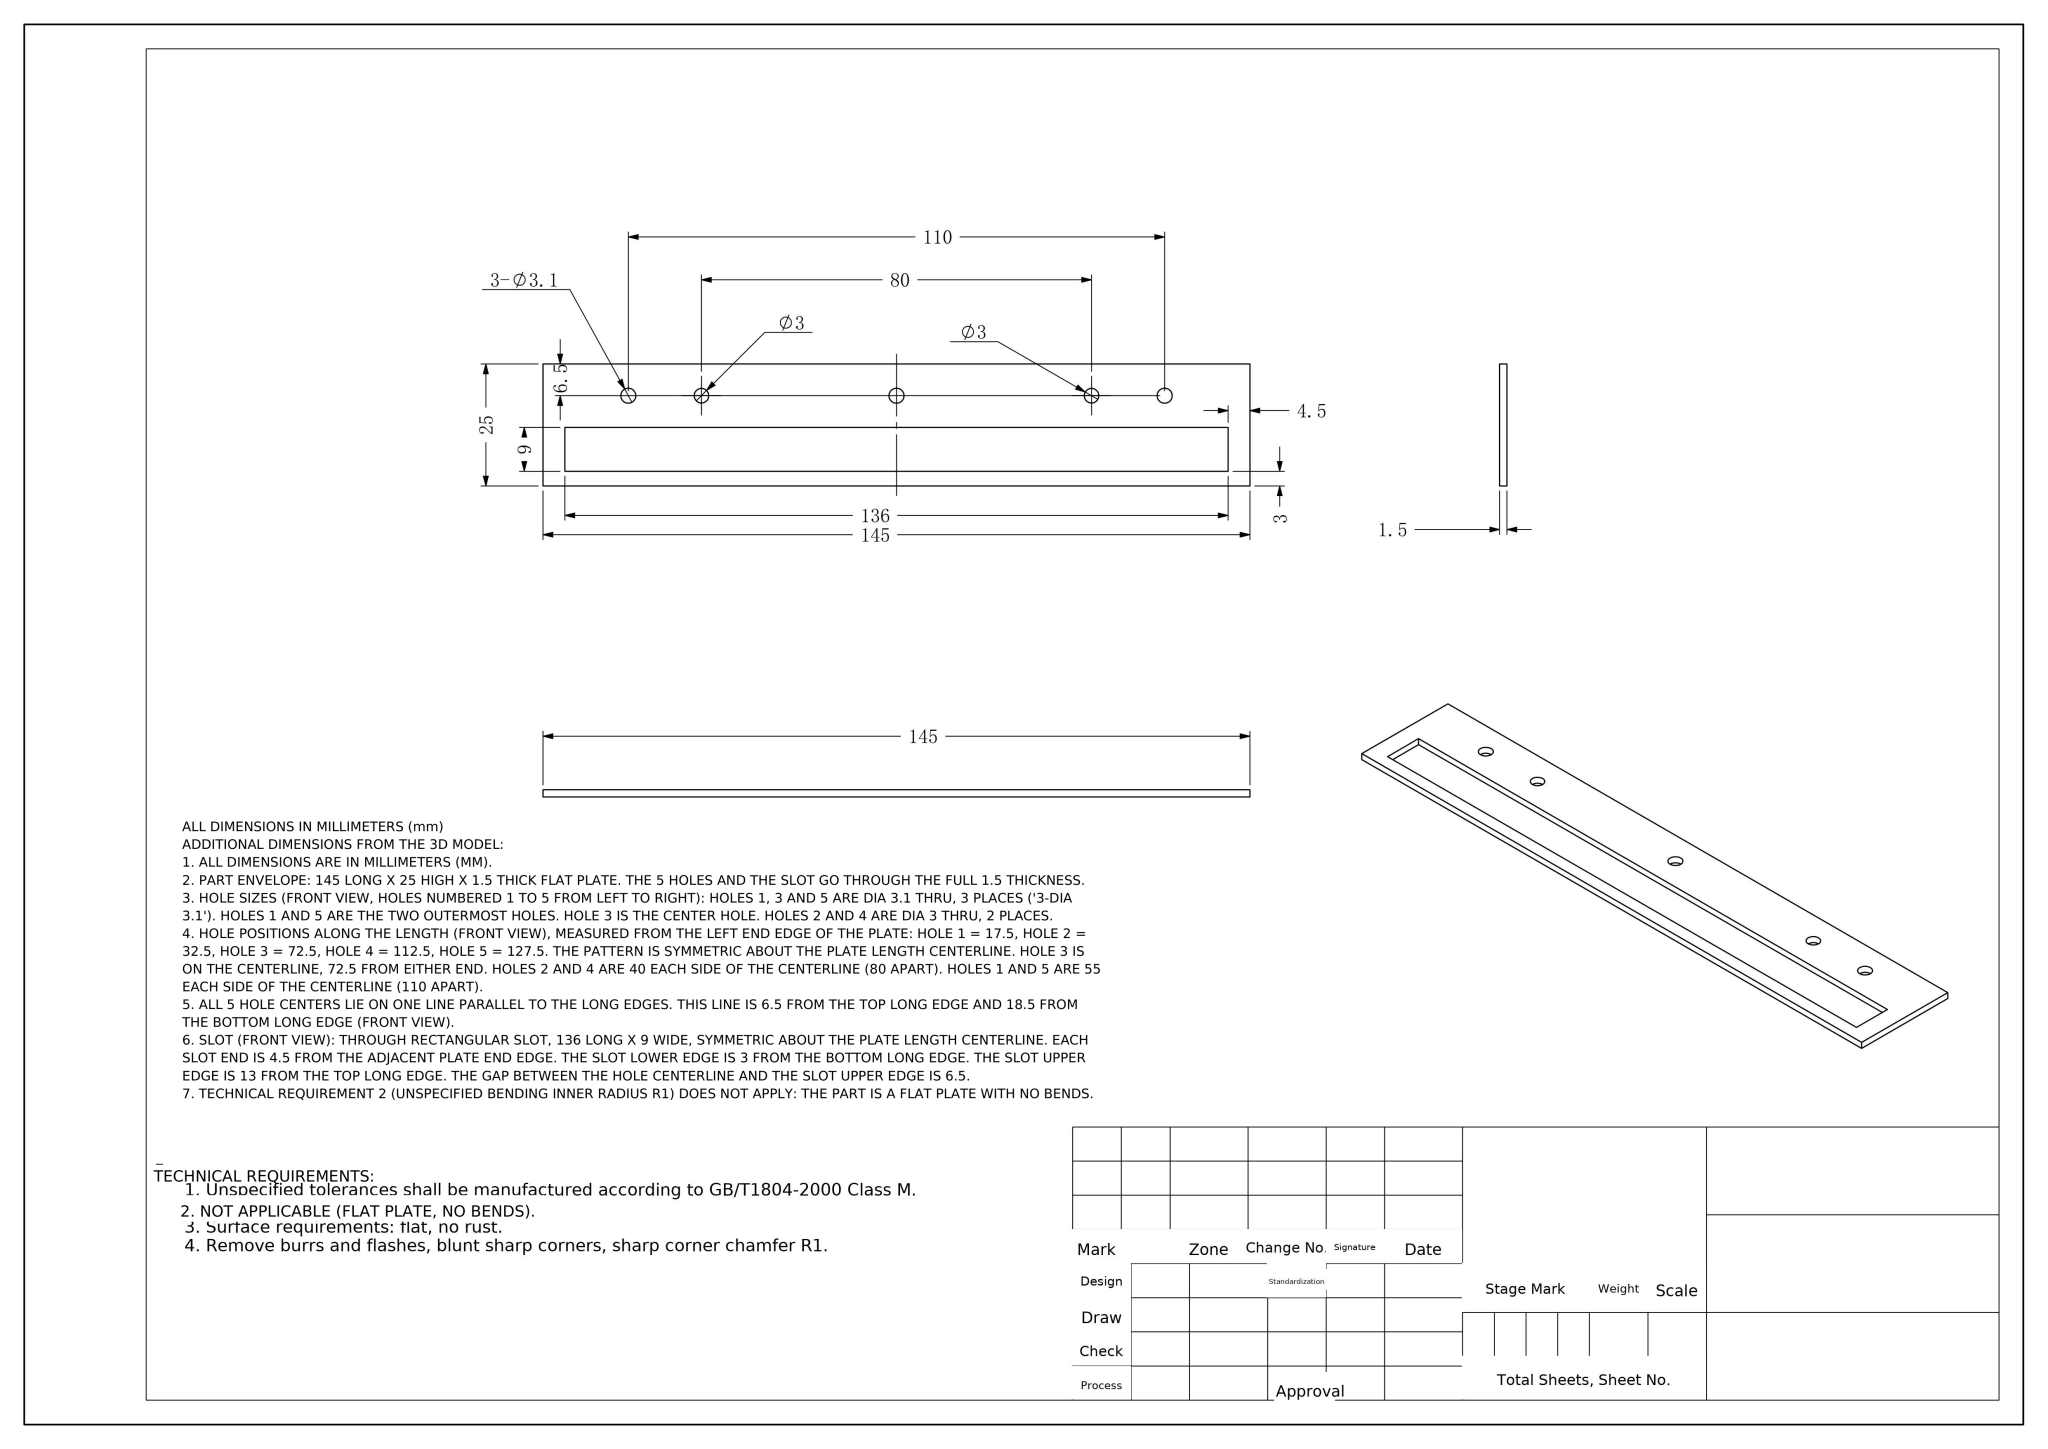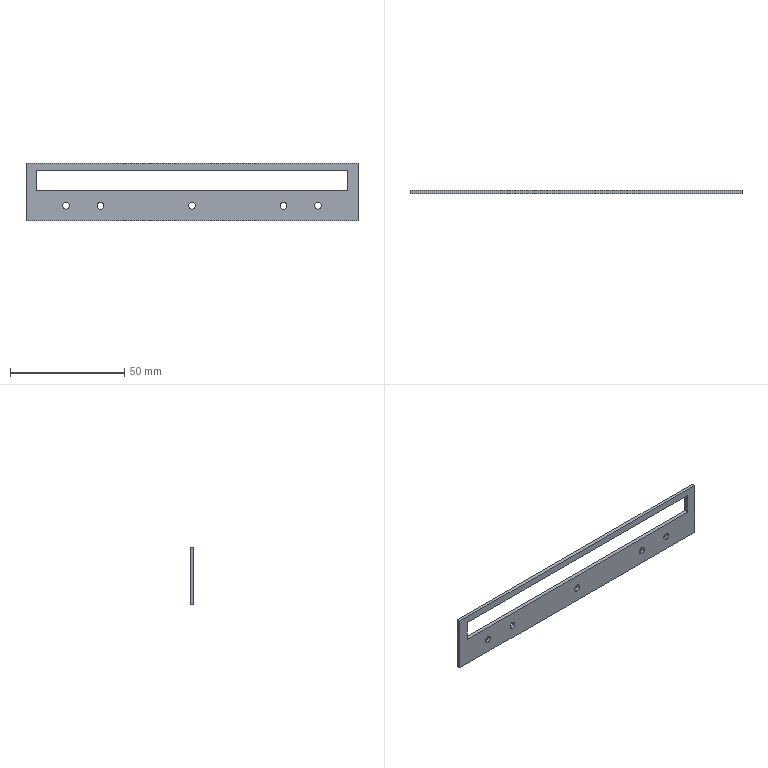Part | NX | mm | 355 | 1 solid | 20 faces | box 145 x 1.5 x 25 mm | volume 3546 mm3 | cylinder 10 | plane 10 | commonest cylinder face diameters 3.1 x6 3 x4
STEP:
#1=COLOUR_RGB('',0.7529,0.7529,0.7529);
#2=FILL_AREA_STYLE_COLOUR('',#1);
#3=FILL_AREA_STYLE('',(#2));
#4=SURFACE_STYLE_FILL_AREA(#3);
#5=SURFACE_SIDE_STYLE('',(#4));
#6=SURFACE_STYLE_USAGE(.BOTH.,#5);
#7=PRESENTATION_STYLE_ASSIGNMENT((#6));
#8=CARTESIAN_POINT('',(55.,-1.5,-7.55));
#9=VERTEX_POINT('',#8);
#10=CARTESIAN_POINT('',(55.,-1.5,-4.45));
#11=VERTEX_POINT('',#10);
#12=CARTESIAN_POINT('',(55.,-1.5,-6.));
#13=DIRECTION('',(0.,1.,0.));
#14=DIRECTION('',(0.,0.,1.));
#15=AXIS2_PLACEMENT_3D('',#12,#13,#14);
#16=CIRCLE('',#15,1.55);
#17=EDGE_CURVE('',#9,#11,#16,.T.);
#18=ORIENTED_EDGE('',*,*,#17,.F.);
#19=CARTESIAN_POINT('',(55.,0.,-7.55));
#20=VERTEX_POINT('',#19);
#21=CARTESIAN_POINT('',(55.,-10.,-7.55));
#22=DIRECTION('',(0.,1.,0.));
#23=VECTOR('',#22,1000.);
#24=LINE('',#21,#23);
#25=EDGE_CURVE('',#9,#20,#24,.T.);
#26=ORIENTED_EDGE('',*,*,#25,.T.);
#27=CARTESIAN_POINT('',(55.,0.,-4.45));
#28=VERTEX_POINT('',#27);
#29=CARTESIAN_POINT('',(55.,0.,-6.));
#30=DIRECTION('',(0.,1.,0.));
#31=DIRECTION('',(0.,0.,1.));
#32=AXIS2_PLACEMENT_3D('',#29,#30,#31);
#33=CIRCLE('',#32,1.55);
#34=EDGE_CURVE('',#20,#28,#33,.T.);
#35=ORIENTED_EDGE('',*,*,#34,.T.);
#36=CARTESIAN_POINT('',(55.,-10.,-4.45));
#37=DIRECTION('',(0.,1.,0.));
#38=VECTOR('',#37,1000.);
#39=LINE('',#36,#38);
#40=EDGE_CURVE('',#11,#28,#39,.T.);
#41=ORIENTED_EDGE('',*,*,#40,.F.);
#42=EDGE_LOOP('',(#18,#26,#35,#41));
#43=FACE_OUTER_BOUND('',#42,.T.);
#44=CARTESIAN_POINT('',(55.,-10.,-6.));
#45=DIRECTION('',(0.,1.,0.));
#46=DIRECTION('',(0.,0.,1.));
#47=AXIS2_PLACEMENT_3D('',#44,#45,#46);
#48=CYLINDRICAL_SURFACE('',#47,1.55);
#49=ADVANCED_FACE('',(#43),#48,.F.);
#50=CARTESIAN_POINT('',(0.,-1.5,-7.55));
#51=VERTEX_POINT('',#50);
#52=CARTESIAN_POINT('',(0.,-1.5,-4.45));
#53=VERTEX_POINT('',#52);
#54=CARTESIAN_POINT('',(0.,-1.5,-6.));
#55=DIRECTION('',(0.,1.,0.));
#56=DIRECTION('',(0.,0.,1.));
#57=AXIS2_PLACEMENT_3D('',#54,#55,#56);
#58=CIRCLE('',#57,1.55);
#59=EDGE_CURVE('',#51,#53,#58,.T.);
#60=ORIENTED_EDGE('',*,*,#59,.F.);
#61=CARTESIAN_POINT('',(0.,0.,-7.55));
#62=VERTEX_POINT('',#61);
#63=CARTESIAN_POINT('',(0.,-10.,-7.55));
#64=DIRECTION('',(0.,1.,0.));
#65=VECTOR('',#64,1000.);
#66=LINE('',#63,#65);
#67=EDGE_CURVE('',#51,#62,#66,.T.);
#68=ORIENTED_EDGE('',*,*,#67,.T.);
#69=CARTESIAN_POINT('',(0.,0.,-4.45));
#70=VERTEX_POINT('',#69);
#71=CARTESIAN_POINT('',(0.,0.,-6.));
#72=DIRECTION('',(0.,1.,0.));
#73=DIRECTION('',(0.,0.,1.));
#74=AXIS2_PLACEMENT_3D('',#71,#72,#73);
#75=CIRCLE('',#74,1.55);
#76=EDGE_CURVE('',#62,#70,#75,.T.);
#77=ORIENTED_EDGE('',*,*,#76,.T.);
#78=CARTESIAN_POINT('',(0.,-10.,-4.45));
#79=DIRECTION('',(0.,1.,0.));
#80=VECTOR('',#79,1000.);
#81=LINE('',#78,#80);
#82=EDGE_CURVE('',#53,#70,#81,.T.);
#83=ORIENTED_EDGE('',*,*,#82,.F.);
#84=EDGE_LOOP('',(#60,#68,#77,#83));
#85=FACE_OUTER_BOUND('',#84,.T.);
#86=CARTESIAN_POINT('',(0.,-10.,-6.));
#87=DIRECTION('',(0.,1.,0.));
#88=DIRECTION('',(0.,0.,1.));
#89=AXIS2_PLACEMENT_3D('',#86,#87,#88);
#90=CYLINDRICAL_SURFACE('',#89,1.55);
#91=ADVANCED_FACE('',(#85),#90,.F.);
#92=CARTESIAN_POINT('',(-55.,-1.5,-7.55));
#93=VERTEX_POINT('',#92);
#94=CARTESIAN_POINT('',(-55.,-1.5,-4.45));
#95=VERTEX_POINT('',#94);
#96=CARTESIAN_POINT('',(-55.,-1.5,-6.));
#97=DIRECTION('',(0.,1.,0.));
#98=DIRECTION('',(0.,0.,1.));
#99=AXIS2_PLACEMENT_3D('',#96,#97,#98);
#100=CIRCLE('',#99,1.55);
#101=EDGE_CURVE('',#93,#95,#100,.T.);
#102=ORIENTED_EDGE('',*,*,#101,.F.);
#103=CARTESIAN_POINT('',(-55.,0.,-7.55));
#104=VERTEX_POINT('',#103);
#105=CARTESIAN_POINT('',(-55.,-10.,-7.55));
#106=DIRECTION('',(0.,1.,0.));
#107=VECTOR('',#106,1000.);
#108=LINE('',#105,#107);
#109=EDGE_CURVE('',#93,#104,#108,.T.);
#110=ORIENTED_EDGE('',*,*,#109,.T.);
#111=CARTESIAN_POINT('',(-55.,0.,-4.45));
#112=VERTEX_POINT('',#111);
#113=CARTESIAN_POINT('',(-55.,0.,-6.));
#114=DIRECTION('',(0.,1.,0.));
#115=DIRECTION('',(0.,0.,1.));
#116=AXIS2_PLACEMENT_3D('',#113,#114,#115);
#117=CIRCLE('',#116,1.55);
#118=EDGE_CURVE('',#104,#112,#117,.T.);
#119=ORIENTED_EDGE('',*,*,#118,.T.);
#120=CARTESIAN_POINT('',(-55.,-10.,-4.45));
#121=DIRECTION('',(0.,1.,0.));
#122=VECTOR('',#121,1000.);
#123=LINE('',#120,#122);
#124=EDGE_CURVE('',#95,#112,#123,.T.);
#125=ORIENTED_EDGE('',*,*,#124,.F.);
#126=EDGE_LOOP('',(#102,#110,#119,#125));
#127=FACE_OUTER_BOUND('',#126,.T.);
#128=CARTESIAN_POINT('',(-55.,-10.,-6.));
#129=DIRECTION('',(0.,1.,0.));
#130=DIRECTION('',(0.,0.,1.));
#131=AXIS2_PLACEMENT_3D('',#128,#129,#130);
#132=CYLINDRICAL_SURFACE('',#131,1.55);
#133=ADVANCED_FACE('',(#127),#132,.F.);
#134=CARTESIAN_POINT('',(-40.,-1.5,-4.5));
#135=VERTEX_POINT('',#134);
#136=CARTESIAN_POINT('',(-40.,-1.5,-7.5));
#137=VERTEX_POINT('',#136);
#138=CARTESIAN_POINT('',(-40.,-1.5,-6.));
#139=DIRECTION('',(0.,-1.,0.));
#140=DIRECTION('',(0.,0.,1.));
#141=AXIS2_PLACEMENT_3D('',#138,#139,#140);
#142=CIRCLE('',#141,1.5);
#143=EDGE_CURVE('',#135,#137,#142,.T.);
#144=ORIENTED_EDGE('',*,*,#143,.T.);
#145=CARTESIAN_POINT('',(-40.,0.,-7.5));
#146=VERTEX_POINT('',#145);
#147=CARTESIAN_POINT('',(-40.,0.,-7.5));
#148=DIRECTION('',(0.,1.,0.));
#149=VECTOR('',#148,1000.);
#150=LINE('',#147,#149);
#151=EDGE_CURVE('',#137,#146,#150,.T.);
#152=ORIENTED_EDGE('',*,*,#151,.T.);
#153=CARTESIAN_POINT('',(-40.,0.,-4.5));
#154=VERTEX_POINT('',#153);
#155=CARTESIAN_POINT('',(-40.,0.,-6.));
#156=DIRECTION('',(0.,-1.,0.));
#157=DIRECTION('',(0.,0.,1.));
#158=AXIS2_PLACEMENT_3D('',#155,#156,#157);
#159=CIRCLE('',#158,1.5);
#160=EDGE_CURVE('',#154,#146,#159,.T.);
#161=ORIENTED_EDGE('',*,*,#160,.F.);
#162=CARTESIAN_POINT('',(-40.,0.,-4.5));
#163=DIRECTION('',(0.,1.,0.));
#164=VECTOR('',#163,1000.);
#165=LINE('',#162,#164);
#166=EDGE_CURVE('',#135,#154,#165,.T.);
#167=ORIENTED_EDGE('',*,*,#166,.F.);
#168=EDGE_LOOP('',(#144,#152,#161,#167));
#169=FACE_OUTER_BOUND('',#168,.T.);
#170=CARTESIAN_POINT('',(-40.,0.,-6.));
#171=DIRECTION('',(0.,1.,0.));
#172=DIRECTION('',(0.,0.,1.));
#173=AXIS2_PLACEMENT_3D('',#170,#171,#172);
#174=CYLINDRICAL_SURFACE('',#173,1.5);
#175=ADVANCED_FACE('',(#169),#174,.F.);
#176=CARTESIAN_POINT('',(40.,-1.5,-4.5));
#177=VERTEX_POINT('',#176);
#178=CARTESIAN_POINT('',(40.,-1.5,-7.5));
#179=VERTEX_POINT('',#178);
#180=CARTESIAN_POINT('',(40.,-1.5,-6.));
#181=DIRECTION('',(0.,-1.,0.));
#182=DIRECTION('',(0.,0.,1.));
#183=AXIS2_PLACEMENT_3D('',#180,#181,#182);
#184=CIRCLE('',#183,1.5);
#185=EDGE_CURVE('',#177,#179,#184,.T.);
#186=ORIENTED_EDGE('',*,*,#185,.T.);
#187=CARTESIAN_POINT('',(40.,0.,-7.5));
#188=VERTEX_POINT('',#187);
#189=CARTESIAN_POINT('',(40.,0.,-7.5));
#190=DIRECTION('',(0.,1.,0.));
#191=VECTOR('',#190,1000.);
#192=LINE('',#189,#191);
#193=EDGE_CURVE('',#179,#188,#192,.T.);
#194=ORIENTED_EDGE('',*,*,#193,.T.);
#195=CARTESIAN_POINT('',(40.,0.,-4.5));
#196=VERTEX_POINT('',#195);
#197=CARTESIAN_POINT('',(40.,0.,-6.));
#198=DIRECTION('',(0.,-1.,0.));
#199=DIRECTION('',(0.,0.,1.));
#200=AXIS2_PLACEMENT_3D('',#197,#198,#199);
#201=CIRCLE('',#200,1.5);
#202=EDGE_CURVE('',#196,#188,#201,.T.);
#203=ORIENTED_EDGE('',*,*,#202,.F.);
#204=CARTESIAN_POINT('',(40.,0.,-4.5));
#205=DIRECTION('',(0.,1.,0.));
#206=VECTOR('',#205,1000.);
#207=LINE('',#204,#206);
#208=EDGE_CURVE('',#177,#196,#207,.T.);
#209=ORIENTED_EDGE('',*,*,#208,.F.);
#210=EDGE_LOOP('',(#186,#194,#203,#209));
#211=FACE_OUTER_BOUND('',#210,.T.);
#212=CARTESIAN_POINT('',(40.,0.,-6.));
#213=DIRECTION('',(0.,1.,0.));
#214=DIRECTION('',(0.,0.,1.));
#215=AXIS2_PLACEMENT_3D('',#212,#213,#214);
#216=CYLINDRICAL_SURFACE('',#215,1.5);
#217=ADVANCED_FACE('',(#211),#216,.F.);
#218=CARTESIAN_POINT('',(-72.5,0.,-12.5));
#219=VERTEX_POINT('',#218);
#220=CARTESIAN_POINT('',(-72.5,0.,12.5));
#221=VERTEX_POINT('',#220);
#222=CARTESIAN_POINT('',(-72.5,0.,-12.5));
#223=DIRECTION('',(0.,0.,1.));
#224=VECTOR('',#223,1000.);
#225=LINE('',#222,#224);
#226=EDGE_CURVE('',#219,#221,#225,.T.);
#227=ORIENTED_EDGE('',*,*,#226,.F.);
#228=CARTESIAN_POINT('',(-72.5,-1.5,-12.5));
#229=VERTEX_POINT('',#228);
#230=CARTESIAN_POINT('',(-72.5,-1.5,-12.5));
#231=DIRECTION('',(0.,1.,0.));
#232=VECTOR('',#231,1000.);
#233=LINE('',#230,#232);
#234=EDGE_CURVE('',#229,#219,#233,.T.);
#235=ORIENTED_EDGE('',*,*,#234,.F.);
#236=CARTESIAN_POINT('',(-72.5,-1.5,12.5));
#237=VERTEX_POINT('',#236);
#238=CARTESIAN_POINT('',(-72.5,-1.5,-12.5));
#239=DIRECTION('',(0.,0.,1.));
#240=VECTOR('',#239,1000.);
#241=LINE('',#238,#240);
#242=EDGE_CURVE('',#229,#237,#241,.T.);
#243=ORIENTED_EDGE('',*,*,#242,.T.);
#244=CARTESIAN_POINT('',(-72.5,-1.5,12.5));
#245=DIRECTION('',(0.,1.,0.));
#246=VECTOR('',#245,1000.);
#247=LINE('',#244,#246);
#248=EDGE_CURVE('',#237,#221,#247,.T.);
#249=ORIENTED_EDGE('',*,*,#248,.T.);
#250=EDGE_LOOP('',(#227,#235,#243,#249));
#251=FACE_OUTER_BOUND('',#250,.T.);
#252=CARTESIAN_POINT('',(-72.5,-1.5,-12.5));
#253=DIRECTION('',(-1.,0.,0.));
#254=DIRECTION('',(0.,0.,1.));
#255=AXIS2_PLACEMENT_3D('',#252,#253,#254);
#256=PLANE('',#255);
#257=ADVANCED_FACE('',(#251),#256,.T.);
#258=CARTESIAN_POINT('',(72.5,0.,12.5));
#259=VERTEX_POINT('',#258);
#260=CARTESIAN_POINT('',(-72.5,0.,12.5));
#261=DIRECTION('',(1.,0.,0.));
#262=VECTOR('',#261,1000.);
#263=LINE('',#260,#262);
#264=EDGE_CURVE('',#221,#259,#263,.T.);
#265=ORIENTED_EDGE('',*,*,#264,.F.);
#266=ORIENTED_EDGE('',*,*,#248,.F.);
#267=CARTESIAN_POINT('',(72.5,-1.5,12.5));
#268=VERTEX_POINT('',#267);
#269=CARTESIAN_POINT('',(-72.5,-1.5,12.5));
#270=DIRECTION('',(1.,0.,0.));
#271=VECTOR('',#270,1000.);
#272=LINE('',#269,#271);
#273=EDGE_CURVE('',#237,#268,#272,.T.);
#274=ORIENTED_EDGE('',*,*,#273,.T.);
#275=CARTESIAN_POINT('',(72.5,-1.5,12.5));
#276=DIRECTION('',(0.,1.,0.));
#277=VECTOR('',#276,1000.);
#278=LINE('',#275,#277);
#279=EDGE_CURVE('',#268,#259,#278,.T.);
#280=ORIENTED_EDGE('',*,*,#279,.T.);
#281=EDGE_LOOP('',(#265,#266,#274,#280));
#282=FACE_OUTER_BOUND('',#281,.T.);
#283=CARTESIAN_POINT('',(-72.5,-1.5,12.5));
#284=DIRECTION('',(0.,0.,1.));
#285=DIRECTION('',(1.,0.,0.));
#286=AXIS2_PLACEMENT_3D('',#283,#284,#285);
#287=PLANE('',#286);
#288=ADVANCED_FACE('',(#282),#287,.T.);
#289=CARTESIAN_POINT('',(72.5,0.,-12.5));
#290=VERTEX_POINT('',#289);
#291=CARTESIAN_POINT('',(72.5,0.,12.5));
#292=DIRECTION('',(0.,0.,-1.));
#293=VECTOR('',#292,1000.);
#294=LINE('',#291,#293);
#295=EDGE_CURVE('',#259,#290,#294,.T.);
#296=ORIENTED_EDGE('',*,*,#295,.F.);
#297=ORIENTED_EDGE('',*,*,#279,.F.);
#298=CARTESIAN_POINT('',(72.5,-1.5,-12.5));
#299=VERTEX_POINT('',#298);
#300=CARTESIAN_POINT('',(72.5,-1.5,12.5));
#301=DIRECTION('',(0.,0.,-1.));
#302=VECTOR('',#301,1000.);
#303=LINE('',#300,#302);
#304=EDGE_CURVE('',#268,#299,#303,.T.);
#305=ORIENTED_EDGE('',*,*,#304,.T.);
#306=CARTESIAN_POINT('',(72.5,-1.5,-12.5));
#307=DIRECTION('',(0.,1.,0.));
#308=VECTOR('',#307,1000.);
#309=LINE('',#306,#308);
#310=EDGE_CURVE('',#299,#290,#309,.T.);
#311=ORIENTED_EDGE('',*,*,#310,.T.);
#312=EDGE_LOOP('',(#296,#297,#305,#311));
#313=FACE_OUTER_BOUND('',#312,.T.);
#314=CARTESIAN_POINT('',(72.5,-1.5,12.5));
#315=DIRECTION('',(1.,0.,0.));
#316=DIRECTION('',(0.,0.,-1.));
#317=AXIS2_PLACEMENT_3D('',#314,#315,#316);
#318=PLANE('',#317);
#319=ADVANCED_FACE('',(#313),#318,.T.);
#320=CARTESIAN_POINT('',(72.5,0.,-12.5));
#321=DIRECTION('',(-1.,0.,-0.));
#322=VECTOR('',#321,1000.);
#323=LINE('',#320,#322);
#324=EDGE_CURVE('',#290,#219,#323,.T.);
#325=ORIENTED_EDGE('',*,*,#324,.F.);
#326=ORIENTED_EDGE('',*,*,#310,.F.);
#327=CARTESIAN_POINT('',(72.5,-1.5,-12.5));
#328=DIRECTION('',(-1.,0.,-0.));
#329=VECTOR('',#328,1000.);
#330=LINE('',#327,#329);
#331=EDGE_CURVE('',#299,#229,#330,.T.);
#332=ORIENTED_EDGE('',*,*,#331,.T.);
#333=ORIENTED_EDGE('',*,*,#234,.T.);
#334=EDGE_LOOP('',(#325,#326,#332,#333));
#335=FACE_OUTER_BOUND('',#334,.T.);
#336=CARTESIAN_POINT('',(72.5,-1.5,-12.5));
#337=DIRECTION('',(0.,0.,-1.));
#338=DIRECTION('',(-1.,0.,-0.));
#339=AXIS2_PLACEMENT_3D('',#336,#337,#338);
#340=PLANE('',#339);
#341=ADVANCED_FACE('',(#335),#340,.T.);
#342=CARTESIAN_POINT('',(55.,-1.5,-6.));
#343=DIRECTION('',(0.,1.,0.));
#344=DIRECTION('',(0.,0.,1.));
#345=AXIS2_PLACEMENT_3D('',#342,#343,#344);
#346=CIRCLE('',#345,1.55);
#347=EDGE_CURVE('',#11,#9,#346,.T.);
#348=ORIENTED_EDGE('',*,*,#347,.T.);
#349=ORIENTED_EDGE('',*,*,#17,.T.);
#350=EDGE_LOOP('',(#348,#349));
#351=FACE_BOUND('',#350,.T.);
#352=CARTESIAN_POINT('',(0.,-1.5,-6.));
#353=DIRECTION('',(0.,1.,0.));
#354=DIRECTION('',(0.,0.,1.));
#355=AXIS2_PLACEMENT_3D('',#352,#353,#354);
#356=CIRCLE('',#355,1.55);
#357=EDGE_CURVE('',#53,#51,#356,.T.);
#358=ORIENTED_EDGE('',*,*,#357,.T.);
#359=ORIENTED_EDGE('',*,*,#59,.T.);
#360=EDGE_LOOP('',(#358,#359));
#361=FACE_BOUND('',#360,.T.);
#362=CARTESIAN_POINT('',(-55.,-1.5,-6.));
#363=DIRECTION('',(0.,1.,0.));
#364=DIRECTION('',(0.,0.,1.));
#365=AXIS2_PLACEMENT_3D('',#362,#363,#364);
#366=CIRCLE('',#365,1.55);
#367=EDGE_CURVE('',#95,#93,#366,.T.);
#368=ORIENTED_EDGE('',*,*,#367,.T.);
#369=ORIENTED_EDGE('',*,*,#101,.T.);
#370=EDGE_LOOP('',(#368,#369));
#371=FACE_BOUND('',#370,.T.);
#372=ORIENTED_EDGE('',*,*,#143,.F.);
#373=CARTESIAN_POINT('',(-40.,-1.5,-6.));
#374=DIRECTION('',(0.,-1.,0.));
#375=DIRECTION('',(0.,0.,1.));
#376=AXIS2_PLACEMENT_3D('',#373,#374,#375);
#377=CIRCLE('',#376,1.5);
#378=EDGE_CURVE('',#137,#135,#377,.T.);
#379=ORIENTED_EDGE('',*,*,#378,.F.);
#380=EDGE_LOOP('',(#372,#379));
#381=FACE_BOUND('',#380,.T.);
#382=ORIENTED_EDGE('',*,*,#185,.F.);
#383=CARTESIAN_POINT('',(40.,-1.5,-6.));
#384=DIRECTION('',(0.,-1.,0.));
#385=DIRECTION('',(0.,0.,1.));
#386=AXIS2_PLACEMENT_3D('',#383,#384,#385);
#387=CIRCLE('',#386,1.5);
#388=EDGE_CURVE('',#179,#177,#387,.T.);
#389=ORIENTED_EDGE('',*,*,#388,.F.);
#390=EDGE_LOOP('',(#382,#389));
#391=FACE_BOUND('',#390,.T.);
#392=CARTESIAN_POINT('',(68.,-1.5,9.5));
#393=VERTEX_POINT('',#392);
#394=CARTESIAN_POINT('',(68.,-1.5,0.5));
#395=VERTEX_POINT('',#394);
#396=CARTESIAN_POINT('',(68.,-1.5,12.5));
#397=DIRECTION('',(0.,0.,-1.));
#398=VECTOR('',#397,1000.);
#399=LINE('',#396,#398);
#400=EDGE_CURVE('',#393,#395,#399,.T.);
#401=ORIENTED_EDGE('',*,*,#400,.T.);
#402=CARTESIAN_POINT('',(-68.,-1.5,0.5));
#403=VERTEX_POINT('',#402);
#404=CARTESIAN_POINT('',(-72.5,-1.5,0.5));
#405=DIRECTION('',(-1.,0.,0.));
#406=VECTOR('',#405,1000.);
#407=LINE('',#404,#406);
#408=EDGE_CURVE('',#395,#403,#407,.T.);
#409=ORIENTED_EDGE('',*,*,#408,.T.);
#410=CARTESIAN_POINT('',(-68.,-1.5,9.5));
#411=VERTEX_POINT('',#410);
#412=CARTESIAN_POINT('',(-68.,-1.5,12.5));
#413=DIRECTION('',(0.,0.,1.));
#414=VECTOR('',#413,1000.);
#415=LINE('',#412,#414);
#416=EDGE_CURVE('',#403,#411,#415,.T.);
#417=ORIENTED_EDGE('',*,*,#416,.T.);
#418=CARTESIAN_POINT('',(-72.5,-1.5,9.5));
#419=DIRECTION('',(1.,0.,0.));
#420=VECTOR('',#419,1000.);
#421=LINE('',#418,#420);
#422=EDGE_CURVE('',#411,#393,#421,.T.);
#423=ORIENTED_EDGE('',*,*,#422,.T.);
#424=EDGE_LOOP('',(#401,#409,#417,#423));
#425=FACE_BOUND('',#424,.T.);
#426=ORIENTED_EDGE('',*,*,#242,.F.);
#427=ORIENTED_EDGE('',*,*,#331,.F.);
#428=ORIENTED_EDGE('',*,*,#304,.F.);
#429=ORIENTED_EDGE('',*,*,#273,.F.);
#430=EDGE_LOOP('',(#426,#427,#428,#429));
#431=FACE_OUTER_BOUND('',#430,.T.);
#432=CARTESIAN_POINT('',(-72.5,-1.5,12.5));
#433=DIRECTION('',(0.,1.,0.));
#434=DIRECTION('',(0.,0.,1.));
#435=AXIS2_PLACEMENT_3D('',#432,#433,#434);
#436=PLANE('',#435);
#437=ADVANCED_FACE('',(#351,#361,#371,#381,#391,#425,#431),#436,.F.);
#438=CARTESIAN_POINT('',(55.,0.,-6.));
#439=DIRECTION('',(0.,1.,0.));
#440=DIRECTION('',(0.,0.,1.));
#441=AXIS2_PLACEMENT_3D('',#438,#439,#440);
#442=CIRCLE('',#441,1.55);
#443=EDGE_CURVE('',#28,#20,#442,.T.);
#444=ORIENTED_EDGE('',*,*,#443,.F.);
#445=ORIENTED_EDGE('',*,*,#34,.F.);
#446=EDGE_LOOP('',(#444,#445));
#447=FACE_BOUND('',#446,.T.);
#448=CARTESIAN_POINT('',(0.,0.,-6.));
#449=DIRECTION('',(0.,1.,0.));
#450=DIRECTION('',(0.,0.,1.));
#451=AXIS2_PLACEMENT_3D('',#448,#449,#450);
#452=CIRCLE('',#451,1.55);
#453=EDGE_CURVE('',#70,#62,#452,.T.);
#454=ORIENTED_EDGE('',*,*,#453,.F.);
#455=ORIENTED_EDGE('',*,*,#76,.F.);
#456=EDGE_LOOP('',(#454,#455));
#457=FACE_BOUND('',#456,.T.);
#458=CARTESIAN_POINT('',(-55.,0.,-6.));
#459=DIRECTION('',(0.,1.,0.));
#460=DIRECTION('',(0.,0.,1.));
#461=AXIS2_PLACEMENT_3D('',#458,#459,#460);
#462=CIRCLE('',#461,1.55);
#463=EDGE_CURVE('',#112,#104,#462,.T.);
#464=ORIENTED_EDGE('',*,*,#463,.F.);
#465=ORIENTED_EDGE('',*,*,#118,.F.);
#466=EDGE_LOOP('',(#464,#465));
#467=FACE_BOUND('',#466,.T.);
#468=ORIENTED_EDGE('',*,*,#160,.T.);
#469=CARTESIAN_POINT('',(-40.,0.,-6.));
#470=DIRECTION('',(0.,-1.,0.));
#471=DIRECTION('',(0.,0.,1.));
#472=AXIS2_PLACEMENT_3D('',#469,#470,#471);
#473=CIRCLE('',#472,1.5);
#474=EDGE_CURVE('',#146,#154,#473,.T.);
#475=ORIENTED_EDGE('',*,*,#474,.T.);
#476=EDGE_LOOP('',(#468,#475));
#477=FACE_BOUND('',#476,.T.);
#478=ORIENTED_EDGE('',*,*,#202,.T.);
#479=CARTESIAN_POINT('',(40.,0.,-6.));
#480=DIRECTION('',(0.,-1.,0.));
#481=DIRECTION('',(0.,0.,1.));
#482=AXIS2_PLACEMENT_3D('',#479,#480,#481);
#483=CIRCLE('',#482,1.5);
#484=EDGE_CURVE('',#188,#196,#483,.T.);
#485=ORIENTED_EDGE('',*,*,#484,.T.);
#486=EDGE_LOOP('',(#478,#485));
#487=FACE_BOUND('',#486,.T.);
#488=CARTESIAN_POINT('',(68.,0.,0.5));
#489=VERTEX_POINT('',#488);
#490=CARTESIAN_POINT('',(-68.,0.,0.5));
#491=VERTEX_POINT('',#490);
#492=CARTESIAN_POINT('',(-72.5,0.,0.5));
#493=DIRECTION('',(-1.,0.,0.));
#494=VECTOR('',#493,1000.);
#495=LINE('',#492,#494);
#496=EDGE_CURVE('',#489,#491,#495,.T.);
#497=ORIENTED_EDGE('',*,*,#496,.F.);
#498=CARTESIAN_POINT('',(68.,0.,9.5));
#499=VERTEX_POINT('',#498);
#500=CARTESIAN_POINT('',(68.,0.,12.5));
#501=DIRECTION('',(0.,0.,-1.));
#502=VECTOR('',#501,1000.);
#503=LINE('',#500,#502);
#504=EDGE_CURVE('',#499,#489,#503,.T.);
#505=ORIENTED_EDGE('',*,*,#504,.F.);
#506=CARTESIAN_POINT('',(-68.,0.,9.5));
#507=VERTEX_POINT('',#506);
#508=CARTESIAN_POINT('',(-72.5,0.,9.5));
#509=DIRECTION('',(1.,0.,0.));
#510=VECTOR('',#509,1000.);
#511=LINE('',#508,#510);
#512=EDGE_CURVE('',#507,#499,#511,.T.);
#513=ORIENTED_EDGE('',*,*,#512,.F.);
#514=CARTESIAN_POINT('',(-68.,0.,12.5));
#515=DIRECTION('',(0.,0.,1.));
#516=VECTOR('',#515,1000.);
#517=LINE('',#514,#516);
#518=EDGE_CURVE('',#491,#507,#517,.T.);
#519=ORIENTED_EDGE('',*,*,#518,.F.);
#520=EDGE_LOOP('',(#497,#505,#513,#519));
#521=FACE_BOUND('',#520,.T.);
#522=ORIENTED_EDGE('',*,*,#226,.T.);
#523=ORIENTED_EDGE('',*,*,#264,.T.);
#524=ORIENTED_EDGE('',*,*,#295,.T.);
#525=ORIENTED_EDGE('',*,*,#324,.T.);
#526=EDGE_LOOP('',(#522,#523,#524,#525));
#527=FACE_OUTER_BOUND('',#526,.T.);
#528=CARTESIAN_POINT('',(-72.5,0.,12.5));
#529=DIRECTION('',(0.,1.,0.));
#530=DIRECTION('',(0.,0.,1.));
#531=AXIS2_PLACEMENT_3D('',#528,#529,#530);
#532=PLANE('',#531);
#533=ADVANCED_FACE('',(#447,#457,#467,#477,#487,#521,#527),#532,.T.);
#534=CARTESIAN_POINT('',(68.,0.,0.5));
#535=DIRECTION('',(0.,1.,0.));
#536=VECTOR('',#535,1000.);
#537=LINE('',#534,#536);
#538=EDGE_CURVE('',#395,#489,#537,.T.);
#539=ORIENTED_EDGE('',*,*,#538,.T.);
#540=ORIENTED_EDGE('',*,*,#496,.T.);
#541=CARTESIAN_POINT('',(-68.,0.,0.5));
#542=DIRECTION('',(0.,1.,0.));
#543=VECTOR('',#542,1000.);
#544=LINE('',#541,#543);
#545=EDGE_CURVE('',#403,#491,#544,.T.);
#546=ORIENTED_EDGE('',*,*,#545,.F.);
#547=ORIENTED_EDGE('',*,*,#408,.F.);
#548=EDGE_LOOP('',(#539,#540,#546,#547));
#549=FACE_OUTER_BOUND('',#548,.T.);
#550=CARTESIAN_POINT('',(-72.5,0.,0.5));
#551=DIRECTION('',(-0.,0.,-1.));
#552=DIRECTION('',(-1.,0.,0.));
#553=AXIS2_PLACEMENT_3D('',#550,#551,#552);
#554=PLANE('',#553);
#555=ADVANCED_FACE('',(#549),#554,.F.);
#556=ORIENTED_EDGE('',*,*,#545,.T.);
#557=ORIENTED_EDGE('',*,*,#518,.T.);
#558=CARTESIAN_POINT('',(-68.,0.,9.5));
#559=DIRECTION('',(0.,1.,0.));
#560=VECTOR('',#559,1000.);
#561=LINE('',#558,#560);
#562=EDGE_CURVE('',#411,#507,#561,.T.);
#563=ORIENTED_EDGE('',*,*,#562,.F.);
#564=ORIENTED_EDGE('',*,*,#416,.F.);
#565=EDGE_LOOP('',(#556,#557,#563,#564));
#566=FACE_OUTER_BOUND('',#565,.T.);
#567=CARTESIAN_POINT('',(-68.,0.,12.5));
#568=DIRECTION('',(-1.,0.,0.));
#569=DIRECTION('',(0.,0.,1.));
#570=AXIS2_PLACEMENT_3D('',#567,#568,#569);
#571=PLANE('',#570);
#572=ADVANCED_FACE('',(#566),#571,.F.);
#573=ORIENTED_EDGE('',*,*,#562,.T.);
#574=ORIENTED_EDGE('',*,*,#512,.T.);
#575=CARTESIAN_POINT('',(68.,0.,9.5));
#576=DIRECTION('',(0.,1.,0.));
#577=VECTOR('',#576,1000.);
#578=LINE('',#575,#577);
#579=EDGE_CURVE('',#393,#499,#578,.T.);
#580=ORIENTED_EDGE('',*,*,#579,.F.);
#581=ORIENTED_EDGE('',*,*,#422,.F.);
#582=EDGE_LOOP('',(#573,#574,#580,#581));
#583=FACE_OUTER_BOUND('',#582,.T.);
#584=CARTESIAN_POINT('',(-72.5,0.,9.5));
#585=DIRECTION('',(0.,0.,1.));
#586=DIRECTION('',(1.,0.,0.));
#587=AXIS2_PLACEMENT_3D('',#584,#585,#586);
#588=PLANE('',#587);
#589=ADVANCED_FACE('',(#583),#588,.F.);
#590=ORIENTED_EDGE('',*,*,#400,.F.);
#591=ORIENTED_EDGE('',*,*,#579,.T.);
#592=ORIENTED_EDGE('',*,*,#504,.T.);
#593=ORIENTED_EDGE('',*,*,#538,.F.);
#594=EDGE_LOOP('',(#590,#591,#592,#593));
#595=FACE_OUTER_BOUND('',#594,.T.);
#596=CARTESIAN_POINT('',(68.,0.,12.5));
#597=DIRECTION('',(1.,0.,0.));
#598=DIRECTION('',(0.,0.,-1.));
#599=AXIS2_PLACEMENT_3D('',#596,#597,#598);
#600=PLANE('',#599);
#601=ADVANCED_FACE('',(#595),#600,.F.);
#602=ORIENTED_EDGE('',*,*,#193,.F.);
#603=ORIENTED_EDGE('',*,*,#388,.T.);
#604=ORIENTED_EDGE('',*,*,#208,.T.);
#605=ORIENTED_EDGE('',*,*,#484,.F.);
#606=EDGE_LOOP('',(#602,#603,#604,#605));
#607=FACE_OUTER_BOUND('',#606,.T.);
#608=CARTESIAN_POINT('',(40.,0.,-6.));
#609=DIRECTION('',(0.,1.,0.));
#610=DIRECTION('',(0.,0.,1.));
#611=AXIS2_PLACEMENT_3D('',#608,#609,#610);
#612=CYLINDRICAL_SURFACE('',#611,1.5);
#613=ADVANCED_FACE('',(#607),#612,.F.);
#614=ORIENTED_EDGE('',*,*,#151,.F.);
#615=ORIENTED_EDGE('',*,*,#378,.T.);
#616=ORIENTED_EDGE('',*,*,#166,.T.);
#617=ORIENTED_EDGE('',*,*,#474,.F.);
#618=EDGE_LOOP('',(#614,#615,#616,#617));
#619=FACE_OUTER_BOUND('',#618,.T.);
#620=CARTESIAN_POINT('',(-40.,0.,-6.));
#621=DIRECTION('',(0.,1.,0.));
#622=DIRECTION('',(0.,0.,1.));
#623=AXIS2_PLACEMENT_3D('',#620,#621,#622);
#624=CYLINDRICAL_SURFACE('',#623,1.5);
#625=ADVANCED_FACE('',(#619),#624,.F.);
#626=ORIENTED_EDGE('',*,*,#109,.F.);
#627=ORIENTED_EDGE('',*,*,#367,.F.);
#628=ORIENTED_EDGE('',*,*,#124,.T.);
#629=ORIENTED_EDGE('',*,*,#463,.T.);
#630=EDGE_LOOP('',(#626,#627,#628,#629));
#631=FACE_OUTER_BOUND('',#630,.T.);
#632=CARTESIAN_POINT('',(-55.,-10.,-6.));
#633=DIRECTION('',(0.,1.,0.));
#634=DIRECTION('',(0.,0.,1.));
#635=AXIS2_PLACEMENT_3D('',#632,#633,#634);
#636=CYLINDRICAL_SURFACE('',#635,1.55);
#637=ADVANCED_FACE('',(#631),#636,.F.);
#638=ORIENTED_EDGE('',*,*,#67,.F.);
#639=ORIENTED_EDGE('',*,*,#357,.F.);
#640=ORIENTED_EDGE('',*,*,#82,.T.);
#641=ORIENTED_EDGE('',*,*,#453,.T.);
#642=EDGE_LOOP('',(#638,#639,#640,#641));
#643=FACE_OUTER_BOUND('',#642,.T.);
#644=CARTESIAN_POINT('',(0.,-10.,-6.));
#645=DIRECTION('',(0.,1.,0.));
#646=DIRECTION('',(0.,0.,1.));
#647=AXIS2_PLACEMENT_3D('',#644,#645,#646);
#648=CYLINDRICAL_SURFACE('',#647,1.55);
#649=ADVANCED_FACE('',(#643),#648,.F.);
#650=ORIENTED_EDGE('',*,*,#25,.F.);
#651=ORIENTED_EDGE('',*,*,#347,.F.);
#652=ORIENTED_EDGE('',*,*,#40,.T.);
#653=ORIENTED_EDGE('',*,*,#443,.T.);
#654=EDGE_LOOP('',(#650,#651,#652,#653));
#655=FACE_OUTER_BOUND('',#654,.T.);
#656=CARTESIAN_POINT('',(55.,-10.,-6.));
#657=DIRECTION('',(0.,1.,0.));
#658=DIRECTION('',(0.,0.,1.));
#659=AXIS2_PLACEMENT_3D('',#656,#657,#658);
#660=CYLINDRICAL_SURFACE('',#659,1.55);
#661=ADVANCED_FACE('',(#655),#660,.F.);
#662=CLOSED_SHELL('',(#49,#91,#133,#175,#217,#257,#288,#319,#341,#437,#533,#555,#572,#589,#601,#613,#625,#637,#649,#661));
#663=MANIFOLD_SOLID_BREP('',#662);
#664=STYLED_ITEM('',(#7),#663);
#665=(LENGTH_UNIT()NAMED_UNIT(*)SI_UNIT(.MILLI.,.METRE.));
#666=UNCERTAINTY_MEASURE_WITH_UNIT(LENGTH_MEASURE(0.00001),#665,'','');
#667=(NAMED_UNIT(*)PLANE_ANGLE_UNIT()SI_UNIT($,.RADIAN.));
#668=(NAMED_UNIT(*)SI_UNIT($,.STERADIAN.)SOLID_ANGLE_UNIT());
#669=(GEOMETRIC_REPRESENTATION_CONTEXT(3)GLOBAL_UNCERTAINTY_ASSIGNED_CONTEXT((#666))GLOBAL_UNIT_ASSIGNED_CONTEXT((#665,#667,#668))REPRESENTATION_CONTEXT('',''));
#670=MECHANICAL_DESIGN_GEOMETRIC_PRESENTATION_REPRESENTATION('',(#664),#669);
#671=PRESENTATION_LAYER_ASSIGNMENT('','',(#664));
#672=COLOUR_RGB('',0.7529,0.7529,0.7529);
#673=FILL_AREA_STYLE_COLOUR('',#672);
#674=FILL_AREA_STYLE('',(#673));
#675=SURFACE_STYLE_FILL_AREA(#674);
#676=SURFACE_SIDE_STYLE('',(#675));
#677=SURFACE_STYLE_USAGE(.BOTH.,#676);
#678=PRESENTATION_STYLE_ASSIGNMENT((#677));
#679=CARTESIAN_POINT('',(0.,0.,0.));
#680=DIRECTION('',(0.,0.,1.));
#681=DIRECTION('',(1.,0.,0.));
#682=AXIS2_PLACEMENT_3D('',#679,#680,#681);
#683=(LENGTH_UNIT()NAMED_UNIT(*)SI_UNIT(.MILLI.,.METRE.));
#684=UNCERTAINTY_MEASURE_WITH_UNIT(LENGTH_MEASURE(0.00001),#683,'','');
#685=(NAMED_UNIT(*)PLANE_ANGLE_UNIT()SI_UNIT($,.RADIAN.));
#686=(NAMED_UNIT(*)SI_UNIT($,.STERADIAN.)SOLID_ANGLE_UNIT());
#687=(GEOMETRIC_REPRESENTATION_CONTEXT(3)GLOBAL_UNCERTAINTY_ASSIGNED_CONTEXT((#684))GLOBAL_UNIT_ASSIGNED_CONTEXT((#683,#685,#686))REPRESENTATION_CONTEXT('',''));
#688=ADVANCED_BREP_SHAPE_REPRESENTATION('',(#663,#682),#687);
#689=STYLED_ITEM('',(#678),#688);
#690=(LENGTH_UNIT()NAMED_UNIT(*)SI_UNIT(.MILLI.,.METRE.));
#691=UNCERTAINTY_MEASURE_WITH_UNIT(LENGTH_MEASURE(0.00001),#690,'','');
#692=(NAMED_UNIT(*)PLANE_ANGLE_UNIT()SI_UNIT($,.RADIAN.));
#693=(NAMED_UNIT(*)SI_UNIT($,.STERADIAN.)SOLID_ANGLE_UNIT());
#694=(GEOMETRIC_REPRESENTATION_CONTEXT(3)GLOBAL_UNCERTAINTY_ASSIGNED_CONTEXT((#691))GLOBAL_UNIT_ASSIGNED_CONTEXT((#690,#692,#693))REPRESENTATION_CONTEXT('',''));
#695=MECHANICAL_DESIGN_GEOMETRIC_PRESENTATION_REPRESENTATION('',(#689),#694);
#696=PRESENTATION_LAYER_ASSIGNMENT('','',(#689));